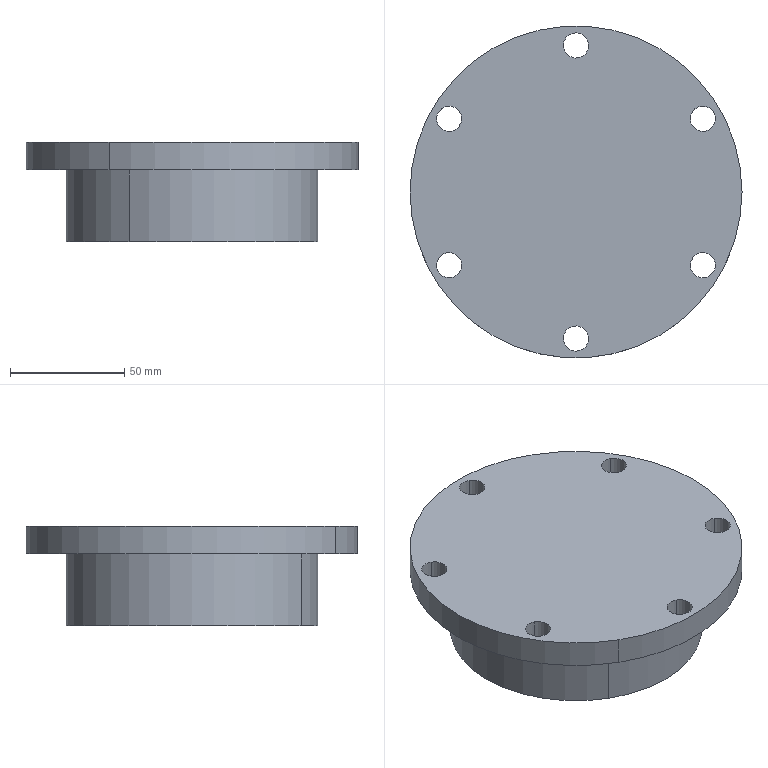Component | SolidWorks | PartAssemblyInLowerHousing-1_FlangeOnWormWheelAxis-2 | 1 solid | 22 faces | box 145 x 145 x 43.25 mm | volume 284628 mm3 | cylinder 16 | plane 4 | cone 2 | commonest cylinder face diameters 11 x12 110 x2 145 x2
build123d program:
from build123d import *

# Parameters (mm, degrees)
SKETCH2_R          = 5.5
CUT_EXTRUDE1_DEPTH = 108.187
CIRPATTERN1_COUNT  = 6
DRAFT1_ANGLE       = 2


with BuildPart() as part:
    # Sketch1 → Revolve1 (revolve)
    with BuildSketch(Plane.XY, mode=Mode.PRIVATE) as revolve1_sk:
        Polygon((0, 0), (0, 72.5), (12, 72.5), (12, 55), (43.25, 55), (43.25, 45), (12, 45), (12, 0), align=None)
    revolve(revolve1_sk.sketch.rotate(Axis((0, 0, 0), (1, 0, 0)), 90), axis=Axis((0, 0, 0), (1, 0, 0)))

    # Sketch2 → Cut-Extrude1 (cut, through all)
    with BuildSketch(Plane(origin=(12, 0, 0), x_dir=(0, 0, -1), z_dir=(1, 0, 0))):
        with Locations((0, 64)):
            Circle(SKETCH2_R)
    cut_extrude1 = extrude(amount=-CUT_EXTRUDE1_DEPTH, mode=Mode.SUBTRACT)

    # CirPattern1: Cut-Extrude1 ×6 about axis
    cirpattern1_axis = Axis((0, 0, 0), (1, 0, 0))
    for i in range(1, CIRPATTERN1_COUNT):
        add(cut_extrude1.rotate(cirpattern1_axis, i * 360 / CIRPATTERN1_COUNT), mode=Mode.SUBTRACT)

    # Draft1
    draft1_faces = [part.faces().sort_by_distance(p)[0] for p in [
        (27.625, 0, -45),
    ]]
    draft(draft1_faces, Plane(origin=(12, 45, 0), x_dir=(0, 0, 1), z_dir=(1, 0, 0)), DRAFT1_ANGLE)


solid = part.part

# Placed as in the assembly
solid = solid.moved(Location((890.83, 1268.591, 1835.217), (0, 90, 0)))
STEP:
#1=COLOUR_RGB('',0.7922,0.8196,0.9333);
#2=FILL_AREA_STYLE_COLOUR('',#1);
#3=FILL_AREA_STYLE('',(#2));
#4=SURFACE_STYLE_FILL_AREA(#3);
#5=SURFACE_SIDE_STYLE('',(#4));
#6=SURFACE_STYLE_USAGE(.BOTH.,#5);
#7=PRESENTATION_STYLE_ASSIGNMENT((#6));
#8=CARTESIAN_POINT('',(32.998,48.872,72.253));
#9=VERTEX_POINT('',#8);
#10=CARTESIAN_POINT('',(32.782,48.497,72.253));
#11=VERTEX_POINT('',#10);
#12=CARTESIAN_POINT('',(32.89,48.685,72.253));
#13=DIRECTION('',(0.,0.,-1.));
#14=DIRECTION('',(0.5,-0.866,0.));
#15=AXIS2_PLACEMENT_3D('',#12,#13,#14);
#16=CIRCLE('',#15,0.2165);
#17=EDGE_CURVE('',#9,#11,#16,.T.);
#18=ORIENTED_EDGE('',*,*,#17,.F.);
#19=CARTESIAN_POINT('',(32.998,48.872,71.78));
#20=VERTEX_POINT('',#19);
#21=CARTESIAN_POINT('',(32.998,48.872,72.253));
#22=DIRECTION('',(0.,0.,-1.));
#23=VECTOR('',#22,39.37);
#24=LINE('',#21,#23);
#25=EDGE_CURVE('',#9,#20,#24,.T.);
#26=ORIENTED_EDGE('',*,*,#25,.T.);
#27=CARTESIAN_POINT('',(32.782,48.497,71.78));
#28=VERTEX_POINT('',#27);
#29=CARTESIAN_POINT('',(32.89,48.685,71.78));
#30=DIRECTION('',(0.,0.,-1.));
#31=DIRECTION('',(0.5,-0.866,0.));
#32=AXIS2_PLACEMENT_3D('',#29,#30,#31);
#33=CIRCLE('',#32,0.2165);
#34=EDGE_CURVE('',#20,#28,#33,.T.);
#35=ORIENTED_EDGE('',*,*,#34,.T.);
#36=CARTESIAN_POINT('',(32.782,48.497,72.253));
#37=DIRECTION('',(0.,0.,-1.));
#38=VECTOR('',#37,39.37);
#39=LINE('',#36,#38);
#40=EDGE_CURVE('',#11,#28,#39,.T.);
#41=ORIENTED_EDGE('',*,*,#40,.F.);
#42=EDGE_LOOP('',(#18,#26,#35,#41));
#43=FACE_OUTER_BOUND('',#42,.T.);
#44=CARTESIAN_POINT('',(32.89,48.685,72.253));
#45=DIRECTION('',(0.,0.,-1.));
#46=DIRECTION('',(-0.5,-0.866,0.));
#47=AXIS2_PLACEMENT_3D('',#44,#45,#46);
#48=CYLINDRICAL_SURFACE('',#47,0.2165);
#49=ADVANCED_FACE('',(#43),#48,.F.);
#50=CARTESIAN_POINT('',(35.18,47.612,72.253));
#51=VERTEX_POINT('',#50);
#52=CARTESIAN_POINT('',(34.964,47.237,72.253));
#53=VERTEX_POINT('',#52);
#54=CARTESIAN_POINT('',(35.072,47.425,72.253));
#55=DIRECTION('',(0.,0.,-1.));
#56=DIRECTION('',(1.,0.,0.));
#57=AXIS2_PLACEMENT_3D('',#54,#55,#56);
#58=CIRCLE('',#57,0.2165);
#59=EDGE_CURVE('',#51,#53,#58,.T.);
#60=ORIENTED_EDGE('',*,*,#59,.F.);
#61=CARTESIAN_POINT('',(35.18,47.612,71.78));
#62=VERTEX_POINT('',#61);
#63=CARTESIAN_POINT('',(35.18,47.612,72.253));
#64=DIRECTION('',(0.,0.,-1.));
#65=VECTOR('',#64,39.37);
#66=LINE('',#63,#65);
#67=EDGE_CURVE('',#51,#62,#66,.T.);
#68=ORIENTED_EDGE('',*,*,#67,.T.);
#69=CARTESIAN_POINT('',(34.964,47.237,71.78));
#70=VERTEX_POINT('',#69);
#71=CARTESIAN_POINT('',(35.072,47.425,71.78));
#72=DIRECTION('',(0.,0.,-1.));
#73=DIRECTION('',(1.,0.,0.));
#74=AXIS2_PLACEMENT_3D('',#71,#72,#73);
#75=CIRCLE('',#74,0.2165);
#76=EDGE_CURVE('',#62,#70,#75,.T.);
#77=ORIENTED_EDGE('',*,*,#76,.T.);
#78=CARTESIAN_POINT('',(34.964,47.237,72.253));
#79=DIRECTION('',(0.,0.,-1.));
#80=VECTOR('',#79,39.37);
#81=LINE('',#78,#80);
#82=EDGE_CURVE('',#53,#70,#81,.T.);
#83=ORIENTED_EDGE('',*,*,#82,.F.);
#84=EDGE_LOOP('',(#60,#68,#77,#83));
#85=FACE_OUTER_BOUND('',#84,.T.);
#86=CARTESIAN_POINT('',(35.072,47.425,72.253));
#87=DIRECTION('',(0.,0.,-1.));
#88=DIRECTION('',(-0.5,-0.866,0.));
#89=AXIS2_PLACEMENT_3D('',#86,#87,#88);
#90=CYLINDRICAL_SURFACE('',#89,0.2165);
#91=ADVANCED_FACE('',(#85),#90,.F.);
#92=CARTESIAN_POINT('',(37.362,48.872,72.253));
#93=VERTEX_POINT('',#92);
#94=CARTESIAN_POINT('',(37.146,48.497,72.253));
#95=VERTEX_POINT('',#94);
#96=CARTESIAN_POINT('',(37.254,48.685,72.253));
#97=DIRECTION('',(0.,0.,-1.));
#98=DIRECTION('',(0.5,0.866,0.));
#99=AXIS2_PLACEMENT_3D('',#96,#97,#98);
#100=CIRCLE('',#99,0.2165);
#101=EDGE_CURVE('',#93,#95,#100,.T.);
#102=ORIENTED_EDGE('',*,*,#101,.F.);
#103=CARTESIAN_POINT('',(37.362,48.872,71.78));
#104=VERTEX_POINT('',#103);
#105=CARTESIAN_POINT('',(37.362,48.872,72.253));
#106=DIRECTION('',(0.,0.,-1.));
#107=VECTOR('',#106,39.37);
#108=LINE('',#105,#107);
#109=EDGE_CURVE('',#93,#104,#108,.T.);
#110=ORIENTED_EDGE('',*,*,#109,.T.);
#111=CARTESIAN_POINT('',(37.146,48.497,71.78));
#112=VERTEX_POINT('',#111);
#113=CARTESIAN_POINT('',(37.254,48.685,71.78));
#114=DIRECTION('',(0.,0.,-1.));
#115=DIRECTION('',(0.5,0.866,0.));
#116=AXIS2_PLACEMENT_3D('',#113,#114,#115);
#117=CIRCLE('',#116,0.2165);
#118=EDGE_CURVE('',#104,#112,#117,.T.);
#119=ORIENTED_EDGE('',*,*,#118,.T.);
#120=CARTESIAN_POINT('',(37.146,48.497,72.253));
#121=DIRECTION('',(0.,0.,-1.));
#122=VECTOR('',#121,39.37);
#123=LINE('',#120,#122);
#124=EDGE_CURVE('',#95,#112,#123,.T.);
#125=ORIENTED_EDGE('',*,*,#124,.F.);
#126=EDGE_LOOP('',(#102,#110,#119,#125));
#127=FACE_OUTER_BOUND('',#126,.T.);
#128=CARTESIAN_POINT('',(37.254,48.685,72.253));
#129=DIRECTION('',(0.,0.,-1.));
#130=DIRECTION('',(-0.5,-0.866,0.));
#131=AXIS2_PLACEMENT_3D('',#128,#129,#130);
#132=CYLINDRICAL_SURFACE('',#131,0.2165);
#133=ADVANCED_FACE('',(#127),#132,.F.);
#134=CARTESIAN_POINT('',(37.362,51.392,72.253));
#135=VERTEX_POINT('',#134);
#136=CARTESIAN_POINT('',(37.146,51.017,72.253));
#137=VERTEX_POINT('',#136);
#138=CARTESIAN_POINT('',(37.254,51.204,72.253));
#139=DIRECTION('',(0.,0.,-1.));
#140=DIRECTION('',(-0.5,0.866,0.));
#141=AXIS2_PLACEMENT_3D('',#138,#139,#140);
#142=CIRCLE('',#141,0.2165);
#143=EDGE_CURVE('',#135,#137,#142,.T.);
#144=ORIENTED_EDGE('',*,*,#143,.F.);
#145=CARTESIAN_POINT('',(37.362,51.392,71.78));
#146=VERTEX_POINT('',#145);
#147=CARTESIAN_POINT('',(37.362,51.392,72.253));
#148=DIRECTION('',(0.,0.,-1.));
#149=VECTOR('',#148,39.37);
#150=LINE('',#147,#149);
#151=EDGE_CURVE('',#135,#146,#150,.T.);
#152=ORIENTED_EDGE('',*,*,#151,.T.);
#153=CARTESIAN_POINT('',(37.146,51.017,71.78));
#154=VERTEX_POINT('',#153);
#155=CARTESIAN_POINT('',(37.254,51.204,71.78));
#156=DIRECTION('',(0.,0.,-1.));
#157=DIRECTION('',(-0.5,0.866,0.));
#158=AXIS2_PLACEMENT_3D('',#155,#156,#157);
#159=CIRCLE('',#158,0.2165);
#160=EDGE_CURVE('',#146,#154,#159,.T.);
#161=ORIENTED_EDGE('',*,*,#160,.T.);
#162=CARTESIAN_POINT('',(37.146,51.017,72.253));
#163=DIRECTION('',(0.,0.,-1.));
#164=VECTOR('',#163,39.37);
#165=LINE('',#162,#164);
#166=EDGE_CURVE('',#137,#154,#165,.T.);
#167=ORIENTED_EDGE('',*,*,#166,.F.);
#168=EDGE_LOOP('',(#144,#152,#161,#167));
#169=FACE_OUTER_BOUND('',#168,.T.);
#170=CARTESIAN_POINT('',(37.254,51.204,72.253));
#171=DIRECTION('',(0.,0.,-1.));
#172=DIRECTION('',(-0.5,-0.866,0.));
#173=AXIS2_PLACEMENT_3D('',#170,#171,#172);
#174=CYLINDRICAL_SURFACE('',#173,0.2165);
#175=ADVANCED_FACE('',(#169),#174,.F.);
#176=CARTESIAN_POINT('',(35.18,52.652,72.253));
#177=VERTEX_POINT('',#176);
#178=CARTESIAN_POINT('',(34.964,52.277,72.253));
#179=VERTEX_POINT('',#178);
#180=CARTESIAN_POINT('',(35.072,52.464,72.253));
#181=DIRECTION('',(0.,0.,-1.));
#182=DIRECTION('',(-1.,0.,0.));
#183=AXIS2_PLACEMENT_3D('',#180,#181,#182);
#184=CIRCLE('',#183,0.2165);
#185=EDGE_CURVE('',#177,#179,#184,.T.);
#186=ORIENTED_EDGE('',*,*,#185,.F.);
#187=CARTESIAN_POINT('',(35.18,52.652,71.78));
#188=VERTEX_POINT('',#187);
#189=CARTESIAN_POINT('',(35.18,52.652,72.253));
#190=DIRECTION('',(0.,0.,-1.));
#191=VECTOR('',#190,39.37);
#192=LINE('',#189,#191);
#193=EDGE_CURVE('',#177,#188,#192,.T.);
#194=ORIENTED_EDGE('',*,*,#193,.T.);
#195=CARTESIAN_POINT('',(34.964,52.277,71.78));
#196=VERTEX_POINT('',#195);
#197=CARTESIAN_POINT('',(35.072,52.464,71.78));
#198=DIRECTION('',(0.,0.,-1.));
#199=DIRECTION('',(-1.,0.,0.));
#200=AXIS2_PLACEMENT_3D('',#197,#198,#199);
#201=CIRCLE('',#200,0.2165);
#202=EDGE_CURVE('',#188,#196,#201,.T.);
#203=ORIENTED_EDGE('',*,*,#202,.T.);
#204=CARTESIAN_POINT('',(34.964,52.277,72.253));
#205=DIRECTION('',(0.,0.,-1.));
#206=VECTOR('',#205,39.37);
#207=LINE('',#204,#206);
#208=EDGE_CURVE('',#179,#196,#207,.T.);
#209=ORIENTED_EDGE('',*,*,#208,.F.);
#210=EDGE_LOOP('',(#186,#194,#203,#209));
#211=FACE_OUTER_BOUND('',#210,.T.);
#212=CARTESIAN_POINT('',(35.072,52.464,72.253));
#213=DIRECTION('',(0.,0.,-1.));
#214=DIRECTION('',(-0.5,-0.866,0.));
#215=AXIS2_PLACEMENT_3D('',#212,#213,#214);
#216=CYLINDRICAL_SURFACE('',#215,0.2165);
#217=ADVANCED_FACE('',(#211),#216,.F.);
#218=CARTESIAN_POINT('',(32.998,51.392,72.253));
#219=VERTEX_POINT('',#218);
#220=CARTESIAN_POINT('',(32.782,51.017,72.253));
#221=VERTEX_POINT('',#220);
#222=CARTESIAN_POINT('',(32.89,51.204,72.253));
#223=DIRECTION('',(0.,0.,-1.));
#224=DIRECTION('',(-0.5,-0.866,0.));
#225=AXIS2_PLACEMENT_3D('',#222,#223,#224);
#226=CIRCLE('',#225,0.2165);
#227=EDGE_CURVE('',#219,#221,#226,.T.);
#228=ORIENTED_EDGE('',*,*,#227,.F.);
#229=CARTESIAN_POINT('',(32.998,51.392,71.78));
#230=VERTEX_POINT('',#229);
#231=CARTESIAN_POINT('',(32.998,51.392,72.253));
#232=DIRECTION('',(0.,0.,-1.));
#233=VECTOR('',#232,39.37);
#234=LINE('',#231,#233);
#235=EDGE_CURVE('',#219,#230,#234,.T.);
#236=ORIENTED_EDGE('',*,*,#235,.T.);
#237=CARTESIAN_POINT('',(32.782,51.017,71.78));
#238=VERTEX_POINT('',#237);
#239=CARTESIAN_POINT('',(32.89,51.204,71.78));
#240=DIRECTION('',(0.,0.,-1.));
#241=DIRECTION('',(-0.5,-0.866,0.));
#242=AXIS2_PLACEMENT_3D('',#239,#240,#241);
#243=CIRCLE('',#242,0.2165);
#244=EDGE_CURVE('',#230,#238,#243,.T.);
#245=ORIENTED_EDGE('',*,*,#244,.T.);
#246=CARTESIAN_POINT('',(32.782,51.017,72.253));
#247=DIRECTION('',(0.,0.,-1.));
#248=VECTOR('',#247,39.37);
#249=LINE('',#246,#248);
#250=EDGE_CURVE('',#221,#238,#249,.T.);
#251=ORIENTED_EDGE('',*,*,#250,.F.);
#252=EDGE_LOOP('',(#228,#236,#245,#251));
#253=FACE_OUTER_BOUND('',#252,.T.);
#254=CARTESIAN_POINT('',(32.89,51.204,72.253));
#255=DIRECTION('',(0.,0.,-1.));
#256=DIRECTION('',(-0.5,-0.866,0.));
#257=AXIS2_PLACEMENT_3D('',#254,#255,#256);
#258=CYLINDRICAL_SURFACE('',#257,0.2165);
#259=ADVANCED_FACE('',(#253),#258,.F.);
#260=CARTESIAN_POINT('',(35.958,51.479,71.78));
#261=VERTEX_POINT('',#260);
#262=CARTESIAN_POINT('',(34.186,48.41,71.78));
#263=VERTEX_POINT('',#262);
#264=CARTESIAN_POINT('',(35.072,49.945,71.78));
#265=DIRECTION('',(0.,0.,1.));
#266=DIRECTION('',(0.5,0.866,0.));
#267=AXIS2_PLACEMENT_3D('',#264,#265,#266);
#268=CIRCLE('',#267,1.772);
#269=EDGE_CURVE('',#261,#263,#268,.T.);
#270=ORIENTED_EDGE('',*,*,#269,.T.);
#271=CARTESIAN_POINT('',(34.165,48.373,70.55));
#272=VERTEX_POINT('',#271);
#273=CARTESIAN_POINT('',(34.186,48.41,71.78));
#274=DIRECTION('',(-0.01745,-0.03022,-0.9994));
#275=VECTOR('',#274,39.37);
#276=LINE('',#273,#275);
#277=EDGE_CURVE('',#263,#272,#276,.T.);
#278=ORIENTED_EDGE('',*,*,#277,.T.);
#279=CARTESIAN_POINT('',(35.979,51.516,70.55));
#280=VERTEX_POINT('',#279);
#281=CARTESIAN_POINT('',(35.072,49.945,70.55));
#282=DIRECTION('',(0.,0.,1.));
#283=DIRECTION('',(0.5,0.866,0.));
#284=AXIS2_PLACEMENT_3D('',#281,#282,#283);
#285=CIRCLE('',#284,1.815);
#286=EDGE_CURVE('',#280,#272,#285,.T.);
#287=ORIENTED_EDGE('',*,*,#286,.F.);
#288=CARTESIAN_POINT('',(35.958,51.479,71.78));
#289=DIRECTION('',(0.01745,0.03022,-0.9994));
#290=VECTOR('',#289,39.37);
#291=LINE('',#288,#290);
#292=EDGE_CURVE('',#261,#280,#291,.T.);
#293=ORIENTED_EDGE('',*,*,#292,.F.);
#294=EDGE_LOOP('',(#270,#278,#287,#293));
#295=FACE_OUTER_BOUND('',#294,.T.);
#296=CARTESIAN_POINT('',(35.072,49.945,71.78));
#297=DIRECTION('',(0.,0.,-1.));
#298=DIRECTION('',(0.5,0.866,0.));
#299=AXIS2_PLACEMENT_3D('',#296,#297,#298);
#300=CONICAL_SURFACE('',#299,1.772,0.03491);
#301=ADVANCED_FACE('',(#295),#300,.F.);
#302=CARTESIAN_POINT('',(36.155,51.82,70.55));
#303=VERTEX_POINT('',#302);
#304=CARTESIAN_POINT('',(33.989,48.069,70.55));
#305=VERTEX_POINT('',#304);
#306=CARTESIAN_POINT('',(35.072,49.945,70.55));
#307=DIRECTION('',(0.,0.,1.));
#308=DIRECTION('',(0.5,0.866,0.));
#309=AXIS2_PLACEMENT_3D('',#306,#307,#308);
#310=CIRCLE('',#309,2.165);
#311=EDGE_CURVE('',#303,#305,#310,.T.);
#312=ORIENTED_EDGE('',*,*,#311,.T.);
#313=CARTESIAN_POINT('',(33.989,48.069,71.78));
#314=VERTEX_POINT('',#313);
#315=CARTESIAN_POINT('',(33.989,48.069,72.253));
#316=DIRECTION('',(0.,0.,1.));
#317=VECTOR('',#316,39.37);
#318=LINE('',#315,#317);
#319=EDGE_CURVE('',#305,#314,#318,.T.);
#320=ORIENTED_EDGE('',*,*,#319,.T.);
#321=CARTESIAN_POINT('',(36.155,51.82,71.78));
#322=VERTEX_POINT('',#321);
#323=CARTESIAN_POINT('',(35.072,49.945,71.78));
#324=DIRECTION('',(0.,0.,1.));
#325=DIRECTION('',(0.5,0.866,0.));
#326=AXIS2_PLACEMENT_3D('',#323,#324,#325);
#327=CIRCLE('',#326,2.165);
#328=EDGE_CURVE('',#322,#314,#327,.T.);
#329=ORIENTED_EDGE('',*,*,#328,.F.);
#330=CARTESIAN_POINT('',(36.155,51.82,72.253));
#331=DIRECTION('',(0.,0.,1.));
#332=VECTOR('',#331,39.37);
#333=LINE('',#330,#332);
#334=EDGE_CURVE('',#303,#322,#333,.T.);
#335=ORIENTED_EDGE('',*,*,#334,.F.);
#336=EDGE_LOOP('',(#312,#320,#329,#335));
#337=FACE_OUTER_BOUND('',#336,.T.);
#338=CARTESIAN_POINT('',(35.072,49.945,72.253));
#339=DIRECTION('',(0.,0.,1.));
#340=DIRECTION('',(0.5,0.866,0.));
#341=AXIS2_PLACEMENT_3D('',#338,#339,#340);
#342=CYLINDRICAL_SURFACE('',#341,2.165);
#343=ADVANCED_FACE('',(#337),#342,.T.);
#344=CARTESIAN_POINT('',(36.499,52.416,71.78));
#345=VERTEX_POINT('',#344);
#346=CARTESIAN_POINT('',(33.645,47.473,71.78));
#347=VERTEX_POINT('',#346);
#348=CARTESIAN_POINT('',(35.072,49.945,71.78));
#349=DIRECTION('',(0.,0.,1.));
#350=DIRECTION('',(0.5,0.866,0.));
#351=AXIS2_PLACEMENT_3D('',#348,#349,#350);
#352=CIRCLE('',#351,2.854);
#353=EDGE_CURVE('',#345,#347,#352,.T.);
#354=ORIENTED_EDGE('',*,*,#353,.T.);
#355=CARTESIAN_POINT('',(33.645,47.473,72.253));
#356=VERTEX_POINT('',#355);
#357=CARTESIAN_POINT('',(33.645,47.473,72.253));
#358=DIRECTION('',(0.,0.,1.));
#359=VECTOR('',#358,39.37);
#360=LINE('',#357,#359);
#361=EDGE_CURVE('',#347,#356,#360,.T.);
#362=ORIENTED_EDGE('',*,*,#361,.T.);
#363=CARTESIAN_POINT('',(36.499,52.416,72.253));
#364=VERTEX_POINT('',#363);
#365=CARTESIAN_POINT('',(35.072,49.945,72.253));
#366=DIRECTION('',(0.,0.,1.));
#367=DIRECTION('',(0.5,0.866,0.));
#368=AXIS2_PLACEMENT_3D('',#365,#366,#367);
#369=CIRCLE('',#368,2.854);
#370=EDGE_CURVE('',#364,#356,#369,.T.);
#371=ORIENTED_EDGE('',*,*,#370,.F.);
#372=CARTESIAN_POINT('',(36.499,52.416,72.253));
#373=DIRECTION('',(0.,0.,1.));
#374=VECTOR('',#373,39.37);
#375=LINE('',#372,#374);
#376=EDGE_CURVE('',#345,#364,#375,.T.);
#377=ORIENTED_EDGE('',*,*,#376,.F.);
#378=EDGE_LOOP('',(#354,#362,#371,#377));
#379=FACE_OUTER_BOUND('',#378,.T.);
#380=CARTESIAN_POINT('',(35.072,49.945,72.253));
#381=DIRECTION('',(0.,0.,1.));
#382=DIRECTION('',(0.5,0.866,0.));
#383=AXIS2_PLACEMENT_3D('',#380,#381,#382);
#384=CYLINDRICAL_SURFACE('',#383,2.854);
#385=ADVANCED_FACE('',(#379),#384,.T.);
#386=CARTESIAN_POINT('',(32.89,48.685,72.253));
#387=DIRECTION('',(0.,0.,-1.));
#388=DIRECTION('',(0.5,-0.866,0.));
#389=AXIS2_PLACEMENT_3D('',#386,#387,#388);
#390=CIRCLE('',#389,0.2165);
#391=EDGE_CURVE('',#11,#9,#390,.T.);
#392=ORIENTED_EDGE('',*,*,#391,.T.);
#393=ORIENTED_EDGE('',*,*,#17,.T.);
#394=EDGE_LOOP('',(#392,#393));
#395=FACE_BOUND('',#394,.T.);
#396=CARTESIAN_POINT('',(35.072,47.425,72.253));
#397=DIRECTION('',(0.,0.,-1.));
#398=DIRECTION('',(1.,0.,0.));
#399=AXIS2_PLACEMENT_3D('',#396,#397,#398);
#400=CIRCLE('',#399,0.2165);
#401=EDGE_CURVE('',#53,#51,#400,.T.);
#402=ORIENTED_EDGE('',*,*,#401,.T.);
#403=ORIENTED_EDGE('',*,*,#59,.T.);
#404=EDGE_LOOP('',(#402,#403));
#405=FACE_BOUND('',#404,.T.);
#406=CARTESIAN_POINT('',(37.254,48.685,72.253));
#407=DIRECTION('',(0.,0.,-1.));
#408=DIRECTION('',(0.5,0.866,0.));
#409=AXIS2_PLACEMENT_3D('',#406,#407,#408);
#410=CIRCLE('',#409,0.2165);
#411=EDGE_CURVE('',#95,#93,#410,.T.);
#412=ORIENTED_EDGE('',*,*,#411,.T.);
#413=ORIENTED_EDGE('',*,*,#101,.T.);
#414=EDGE_LOOP('',(#412,#413));
#415=FACE_BOUND('',#414,.T.);
#416=CARTESIAN_POINT('',(37.254,51.204,72.253));
#417=DIRECTION('',(0.,0.,-1.));
#418=DIRECTION('',(-0.5,0.866,0.));
#419=AXIS2_PLACEMENT_3D('',#416,#417,#418);
#420=CIRCLE('',#419,0.2165);
#421=EDGE_CURVE('',#137,#135,#420,.T.);
#422=ORIENTED_EDGE('',*,*,#421,.T.);
#423=ORIENTED_EDGE('',*,*,#143,.T.);
#424=EDGE_LOOP('',(#422,#423));
#425=FACE_BOUND('',#424,.T.);
#426=CARTESIAN_POINT('',(35.072,52.464,72.253));
#427=DIRECTION('',(0.,0.,-1.));
#428=DIRECTION('',(-1.,0.,0.));
#429=AXIS2_PLACEMENT_3D('',#426,#427,#428);
#430=CIRCLE('',#429,0.2165);
#431=EDGE_CURVE('',#179,#177,#430,.T.);
#432=ORIENTED_EDGE('',*,*,#431,.T.);
#433=ORIENTED_EDGE('',*,*,#185,.T.);
#434=EDGE_LOOP('',(#432,#433));
#435=FACE_BOUND('',#434,.T.);
#436=CARTESIAN_POINT('',(32.89,51.204,72.253));
#437=DIRECTION('',(0.,0.,-1.));
#438=DIRECTION('',(-0.5,-0.866,0.));
#439=AXIS2_PLACEMENT_3D('',#436,#437,#438);
#440=CIRCLE('',#439,0.2165);
#441=EDGE_CURVE('',#221,#219,#440,.T.);
#442=ORIENTED_EDGE('',*,*,#441,.T.);
#443=ORIENTED_EDGE('',*,*,#227,.T.);
#444=EDGE_LOOP('',(#442,#443));
#445=FACE_BOUND('',#444,.T.);
#446=ORIENTED_EDGE('',*,*,#370,.T.);
#447=CARTESIAN_POINT('',(35.072,49.945,72.253));
#448=DIRECTION('',(0.,0.,1.));
#449=DIRECTION('',(0.5,0.866,0.));
#450=AXIS2_PLACEMENT_3D('',#447,#448,#449);
#451=CIRCLE('',#450,2.854);
#452=EDGE_CURVE('',#356,#364,#451,.T.);
#453=ORIENTED_EDGE('',*,*,#452,.T.);
#454=EDGE_LOOP('',(#446,#453));
#455=FACE_OUTER_BOUND('',#454,.T.);
#456=CARTESIAN_POINT('',(35.072,49.945,72.253));
#457=DIRECTION('',(0.,0.,-1.));
#458=DIRECTION('',(-0.5,-0.866,0.));
#459=AXIS2_PLACEMENT_3D('',#456,#457,#458);
#460=PLANE('',#459);
#461=ADVANCED_FACE('',(#395,#405,#415,#425,#435,#445,#455),#460,.F.);
#462=ORIENTED_EDGE('',*,*,#361,.F.);
#463=CARTESIAN_POINT('',(35.072,49.945,71.78));
#464=DIRECTION('',(0.,0.,1.));
#465=DIRECTION('',(0.5,0.866,0.));
#466=AXIS2_PLACEMENT_3D('',#463,#464,#465);
#467=CIRCLE('',#466,2.854);
#468=EDGE_CURVE('',#347,#345,#467,.T.);
#469=ORIENTED_EDGE('',*,*,#468,.T.);
#470=ORIENTED_EDGE('',*,*,#376,.T.);
#471=ORIENTED_EDGE('',*,*,#452,.F.);
#472=EDGE_LOOP('',(#462,#469,#470,#471));
#473=FACE_OUTER_BOUND('',#472,.T.);
#474=CARTESIAN_POINT('',(35.072,49.945,72.253));
#475=DIRECTION('',(0.,0.,1.));
#476=DIRECTION('',(0.5,0.866,0.));
#477=AXIS2_PLACEMENT_3D('',#474,#475,#476);
#478=CYLINDRICAL_SURFACE('',#477,2.854);
#479=ADVANCED_FACE('',(#473),#478,.T.);
#480=CARTESIAN_POINT('',(32.89,48.685,71.78));
#481=DIRECTION('',(0.,0.,-1.));
#482=DIRECTION('',(0.5,-0.866,0.));
#483=AXIS2_PLACEMENT_3D('',#480,#481,#482);
#484=CIRCLE('',#483,0.2165);
#485=EDGE_CURVE('',#28,#20,#484,.T.);
#486=ORIENTED_EDGE('',*,*,#485,.F.);
#487=ORIENTED_EDGE('',*,*,#34,.F.);
#488=EDGE_LOOP('',(#486,#487));
#489=FACE_BOUND('',#488,.T.);
#490=CARTESIAN_POINT('',(35.072,47.425,71.78));
#491=DIRECTION('',(0.,0.,-1.));
#492=DIRECTION('',(1.,0.,0.));
#493=AXIS2_PLACEMENT_3D('',#490,#491,#492);
#494=CIRCLE('',#493,0.2165);
#495=EDGE_CURVE('',#70,#62,#494,.T.);
#496=ORIENTED_EDGE('',*,*,#495,.F.);
#497=ORIENTED_EDGE('',*,*,#76,.F.);
#498=EDGE_LOOP('',(#496,#497));
#499=FACE_BOUND('',#498,.T.);
#500=CARTESIAN_POINT('',(37.254,48.685,71.78));
#501=DIRECTION('',(0.,0.,-1.));
#502=DIRECTION('',(0.5,0.866,0.));
#503=AXIS2_PLACEMENT_3D('',#500,#501,#502);
#504=CIRCLE('',#503,0.2165);
#505=EDGE_CURVE('',#112,#104,#504,.T.);
#506=ORIENTED_EDGE('',*,*,#505,.F.);
#507=ORIENTED_EDGE('',*,*,#118,.F.);
#508=EDGE_LOOP('',(#506,#507));
#509=FACE_BOUND('',#508,.T.);
#510=CARTESIAN_POINT('',(37.254,51.204,71.78));
#511=DIRECTION('',(0.,0.,-1.));
#512=DIRECTION('',(-0.5,0.866,0.));
#513=AXIS2_PLACEMENT_3D('',#510,#511,#512);
#514=CIRCLE('',#513,0.2165);
#515=EDGE_CURVE('',#154,#146,#514,.T.);
#516=ORIENTED_EDGE('',*,*,#515,.F.);
#517=ORIENTED_EDGE('',*,*,#160,.F.);
#518=EDGE_LOOP('',(#516,#517));
#519=FACE_BOUND('',#518,.T.);
#520=CARTESIAN_POINT('',(35.072,52.464,71.78));
#521=DIRECTION('',(0.,0.,-1.));
#522=DIRECTION('',(-1.,0.,0.));
#523=AXIS2_PLACEMENT_3D('',#520,#521,#522);
#524=CIRCLE('',#523,0.2165);
#525=EDGE_CURVE('',#196,#188,#524,.T.);
#526=ORIENTED_EDGE('',*,*,#525,.F.);
#527=ORIENTED_EDGE('',*,*,#202,.F.);
#528=EDGE_LOOP('',(#526,#527));
#529=FACE_BOUND('',#528,.T.);
#530=CARTESIAN_POINT('',(32.89,51.204,71.78));
#531=DIRECTION('',(0.,0.,-1.));
#532=DIRECTION('',(-0.5,-0.866,0.));
#533=AXIS2_PLACEMENT_3D('',#530,#531,#532);
#534=CIRCLE('',#533,0.2165);
#535=EDGE_CURVE('',#238,#230,#534,.T.);
#536=ORIENTED_EDGE('',*,*,#535,.F.);
#537=ORIENTED_EDGE('',*,*,#244,.F.);
#538=EDGE_LOOP('',(#536,#537));
#539=FACE_BOUND('',#538,.T.);
#540=ORIENTED_EDGE('',*,*,#353,.F.);
#541=ORIENTED_EDGE('',*,*,#468,.F.);
#542=EDGE_LOOP('',(#540,#541));
#543=FACE_OUTER_BOUND('',#542,.T.);
#544=ORIENTED_EDGE('',*,*,#328,.T.);
#545=CARTESIAN_POINT('',(35.072,49.945,71.78));
#546=DIRECTION('',(0.,0.,1.));
#547=DIRECTION('',(0.5,0.866,0.));
#548=AXIS2_PLACEMENT_3D('',#545,#546,#547);
#549=CIRCLE('',#548,2.165);
#550=EDGE_CURVE('',#314,#322,#549,.T.);
#551=ORIENTED_EDGE('',*,*,#550,.T.);
#552=EDGE_LOOP('',(#544,#551));
#553=FACE_BOUND('',#552,.T.);
#554=CARTESIAN_POINT('',(32.6,51.372,71.78));
#555=DIRECTION('',(0.,0.,1.));
#556=DIRECTION('',(0.5,0.866,0.));
#557=AXIS2_PLACEMENT_3D('',#554,#555,#556);
#558=PLANE('',#557);
#559=ADVANCED_FACE('',(#489,#499,#509,#519,#529,#539,#543,#553),#558,.F.);
#560=ORIENTED_EDGE('',*,*,#319,.F.);
#561=CARTESIAN_POINT('',(35.072,49.945,70.55));
#562=DIRECTION('',(0.,0.,1.));
#563=DIRECTION('',(0.5,0.866,0.));
#564=AXIS2_PLACEMENT_3D('',#561,#562,#563);
#565=CIRCLE('',#564,2.165);
#566=EDGE_CURVE('',#305,#303,#565,.T.);
#567=ORIENTED_EDGE('',*,*,#566,.T.);
#568=ORIENTED_EDGE('',*,*,#334,.T.);
#569=ORIENTED_EDGE('',*,*,#550,.F.);
#570=EDGE_LOOP('',(#560,#567,#568,#569));
#571=FACE_OUTER_BOUND('',#570,.T.);
#572=CARTESIAN_POINT('',(35.072,49.945,72.253));
#573=DIRECTION('',(0.,0.,1.));
#574=DIRECTION('',(0.5,0.866,0.));
#575=AXIS2_PLACEMENT_3D('',#572,#573,#574);
#576=CYLINDRICAL_SURFACE('',#575,2.165);
#577=ADVANCED_FACE('',(#571),#576,.T.);
#578=ORIENTED_EDGE('',*,*,#311,.F.);
#579=ORIENTED_EDGE('',*,*,#566,.F.);
#580=EDGE_LOOP('',(#578,#579));
#581=FACE_OUTER_BOUND('',#580,.T.);
#582=ORIENTED_EDGE('',*,*,#286,.T.);
#583=CARTESIAN_POINT('',(35.072,49.945,70.55));
#584=DIRECTION('',(0.,0.,1.));
#585=DIRECTION('',(0.5,0.866,0.));
#586=AXIS2_PLACEMENT_3D('',#583,#584,#585);
#587=CIRCLE('',#586,1.815);
#588=EDGE_CURVE('',#272,#280,#587,.T.);
#589=ORIENTED_EDGE('',*,*,#588,.T.);
#590=EDGE_LOOP('',(#582,#589));
#591=FACE_BOUND('',#590,.T.);
#592=CARTESIAN_POINT('',(33.197,51.027,70.55));
#593=DIRECTION('',(0.,0.,1.));
#594=DIRECTION('',(0.5,0.866,0.));
#595=AXIS2_PLACEMENT_3D('',#592,#593,#594);
#596=PLANE('',#595);
#597=ADVANCED_FACE('',(#581,#591),#596,.F.);
#598=ORIENTED_EDGE('',*,*,#277,.F.);
#599=CARTESIAN_POINT('',(35.072,49.945,71.78));
#600=DIRECTION('',(0.,0.,1.));
#601=DIRECTION('',(0.5,0.866,0.));
#602=AXIS2_PLACEMENT_3D('',#599,#600,#601);
#603=CIRCLE('',#602,1.772);
#604=EDGE_CURVE('',#263,#261,#603,.T.);
#605=ORIENTED_EDGE('',*,*,#604,.T.);
#606=ORIENTED_EDGE('',*,*,#292,.T.);
#607=ORIENTED_EDGE('',*,*,#588,.F.);
#608=EDGE_LOOP('',(#598,#605,#606,#607));
#609=FACE_OUTER_BOUND('',#608,.T.);
#610=CARTESIAN_POINT('',(35.072,49.945,71.78));
#611=DIRECTION('',(0.,0.,-1.));
#612=DIRECTION('',(0.5,0.866,0.));
#613=AXIS2_PLACEMENT_3D('',#610,#611,#612);
#614=CONICAL_SURFACE('',#613,1.772,0.03491);
#615=ADVANCED_FACE('',(#609),#614,.F.);
#616=ORIENTED_EDGE('',*,*,#269,.F.);
#617=ORIENTED_EDGE('',*,*,#604,.F.);
#618=EDGE_LOOP('',(#616,#617));
#619=FACE_OUTER_BOUND('',#618,.T.);
#620=CARTESIAN_POINT('',(33.538,50.83,71.78));
#621=DIRECTION('',(0.,0.,1.));
#622=DIRECTION('',(0.5,0.866,0.));
#623=AXIS2_PLACEMENT_3D('',#620,#621,#622);
#624=PLANE('',#623);
#625=ADVANCED_FACE('',(#619),#624,.F.);
#626=ORIENTED_EDGE('',*,*,#235,.F.);
#627=ORIENTED_EDGE('',*,*,#441,.F.);
#628=ORIENTED_EDGE('',*,*,#250,.T.);
#629=ORIENTED_EDGE('',*,*,#535,.T.);
#630=EDGE_LOOP('',(#626,#627,#628,#629));
#631=FACE_OUTER_BOUND('',#630,.T.);
#632=CARTESIAN_POINT('',(32.89,51.204,72.253));
#633=DIRECTION('',(0.,0.,-1.));
#634=DIRECTION('',(-0.5,-0.866,0.));
#635=AXIS2_PLACEMENT_3D('',#632,#633,#634);
#636=CYLINDRICAL_SURFACE('',#635,0.2165);
#637=ADVANCED_FACE('',(#631),#636,.F.);
#638=ORIENTED_EDGE('',*,*,#193,.F.);
#639=ORIENTED_EDGE('',*,*,#431,.F.);
#640=ORIENTED_EDGE('',*,*,#208,.T.);
#641=ORIENTED_EDGE('',*,*,#525,.T.);
#642=EDGE_LOOP('',(#638,#639,#640,#641));
#643=FACE_OUTER_BOUND('',#642,.T.);
#644=CARTESIAN_POINT('',(35.072,52.464,72.253));
#645=DIRECTION('',(0.,0.,-1.));
#646=DIRECTION('',(-0.5,-0.866,0.));
#647=AXIS2_PLACEMENT_3D('',#644,#645,#646);
#648=CYLINDRICAL_SURFACE('',#647,0.2165);
#649=ADVANCED_FACE('',(#643),#648,.F.);
#650=ORIENTED_EDGE('',*,*,#151,.F.);
#651=ORIENTED_EDGE('',*,*,#421,.F.);
#652=ORIENTED_EDGE('',*,*,#166,.T.);
#653=ORIENTED_EDGE('',*,*,#515,.T.);
#654=EDGE_LOOP('',(#650,#651,#652,#653));
#655=FACE_OUTER_BOUND('',#654,.T.);
#656=CARTESIAN_POINT('',(37.254,51.204,72.253));
#657=DIRECTION('',(0.,0.,-1.));
#658=DIRECTION('',(-0.5,-0.866,0.));
#659=AXIS2_PLACEMENT_3D('',#656,#657,#658);
#660=CYLINDRICAL_SURFACE('',#659,0.2165);
#661=ADVANCED_FACE('',(#655),#660,.F.);
#662=ORIENTED_EDGE('',*,*,#109,.F.);
#663=ORIENTED_EDGE('',*,*,#411,.F.);
#664=ORIENTED_EDGE('',*,*,#124,.T.);
#665=ORIENTED_EDGE('',*,*,#505,.T.);
#666=EDGE_LOOP('',(#662,#663,#664,#665));
#667=FACE_OUTER_BOUND('',#666,.T.);
#668=CARTESIAN_POINT('',(37.254,48.685,72.253));
#669=DIRECTION('',(0.,0.,-1.));
#670=DIRECTION('',(-0.5,-0.866,0.));
#671=AXIS2_PLACEMENT_3D('',#668,#669,#670);
#672=CYLINDRICAL_SURFACE('',#671,0.2165);
#673=ADVANCED_FACE('',(#667),#672,.F.);
#674=ORIENTED_EDGE('',*,*,#67,.F.);
#675=ORIENTED_EDGE('',*,*,#401,.F.);
#676=ORIENTED_EDGE('',*,*,#82,.T.);
#677=ORIENTED_EDGE('',*,*,#495,.T.);
#678=EDGE_LOOP('',(#674,#675,#676,#677));
#679=FACE_OUTER_BOUND('',#678,.T.);
#680=CARTESIAN_POINT('',(35.072,47.425,72.253));
#681=DIRECTION('',(0.,0.,-1.));
#682=DIRECTION('',(-0.5,-0.866,0.));
#683=AXIS2_PLACEMENT_3D('',#680,#681,#682);
#684=CYLINDRICAL_SURFACE('',#683,0.2165);
#685=ADVANCED_FACE('',(#679),#684,.F.);
#686=ORIENTED_EDGE('',*,*,#25,.F.);
#687=ORIENTED_EDGE('',*,*,#391,.F.);
#688=ORIENTED_EDGE('',*,*,#40,.T.);
#689=ORIENTED_EDGE('',*,*,#485,.T.);
#690=EDGE_LOOP('',(#686,#687,#688,#689));
#691=FACE_OUTER_BOUND('',#690,.T.);
#692=CARTESIAN_POINT('',(32.89,48.685,72.253));
#693=DIRECTION('',(0.,0.,-1.));
#694=DIRECTION('',(-0.5,-0.866,0.));
#695=AXIS2_PLACEMENT_3D('',#692,#693,#694);
#696=CYLINDRICAL_SURFACE('',#695,0.2165);
#697=ADVANCED_FACE('',(#691),#696,.F.);
#698=CLOSED_SHELL('',(#49,#91,#133,#175,#217,#259,#301,#343,#385,#461,#479,#559,#577,#597,#615,#625,#637,#649,#661,#673,#685,#697));
#699=MANIFOLD_SOLID_BREP('',#698);
#700=STYLED_ITEM('',(#7),#699);
#701=PRESENTATION_LAYER_ASSIGNMENT('','',(#700));
#702=CARTESIAN_POINT('',(0.,0.,0.));
#703=DIRECTION('',(0.,0.,1.));
#704=DIRECTION('',(1.,0.,0.));
#705=AXIS2_PLACEMENT_3D('',#702,#703,#704);
#706=(LENGTH_UNIT()NAMED_UNIT(*)SI_UNIT($,.METRE.));
#707=LENGTH_MEASURE_WITH_UNIT(LENGTH_MEASURE(0.0254),#706);
#708=DIMENSIONAL_EXPONENTS(1.,0.,0.,0.,0.,0.,0.);
#709=(CONVERSION_BASED_UNIT('',#707)LENGTH_UNIT()NAMED_UNIT(#708));
#710=UNCERTAINTY_MEASURE_WITH_UNIT(LENGTH_MEASURE(0.00001),#709,'','');
#711=(NAMED_UNIT(*)PLANE_ANGLE_UNIT()SI_UNIT($,.RADIAN.));
#712=(NAMED_UNIT(*)SI_UNIT($,.STERADIAN.)SOLID_ANGLE_UNIT());
#713=(GEOMETRIC_REPRESENTATION_CONTEXT(3)GLOBAL_UNCERTAINTY_ASSIGNED_CONTEXT((#710))GLOBAL_UNIT_ASSIGNED_CONTEXT((#709,#711,#712))REPRESENTATION_CONTEXT('',''));
#714=ADVANCED_BREP_SHAPE_REPRESENTATION('',(#699,#705),#713);
#715=(LENGTH_UNIT()NAMED_UNIT(*)SI_UNIT($,.METRE.));
#716=LENGTH_MEASURE_WITH_UNIT(LENGTH_MEASURE(0.0254),#715);
#717=DIMENSIONAL_EXPONENTS(1.,0.,0.,0.,0.,0.,0.);
#718=(CONVERSION_BASED_UNIT('',#716)LENGTH_UNIT()NAMED_UNIT(#717));
#719=UNCERTAINTY_MEASURE_WITH_UNIT(LENGTH_MEASURE(0.00001),#718,'','');
#720=(NAMED_UNIT(*)PLANE_ANGLE_UNIT()SI_UNIT($,.RADIAN.));
#721=(NAMED_UNIT(*)SI_UNIT($,.STERADIAN.)SOLID_ANGLE_UNIT());
#722=(GEOMETRIC_REPRESENTATION_CONTEXT(3)GLOBAL_UNCERTAINTY_ASSIGNED_CONTEXT((#719))GLOBAL_UNIT_ASSIGNED_CONTEXT((#718,#720,#721))REPRESENTATION_CONTEXT('',''));
#723=MECHANICAL_DESIGN_GEOMETRIC_PRESENTATION_REPRESENTATION('',(#700),#722);